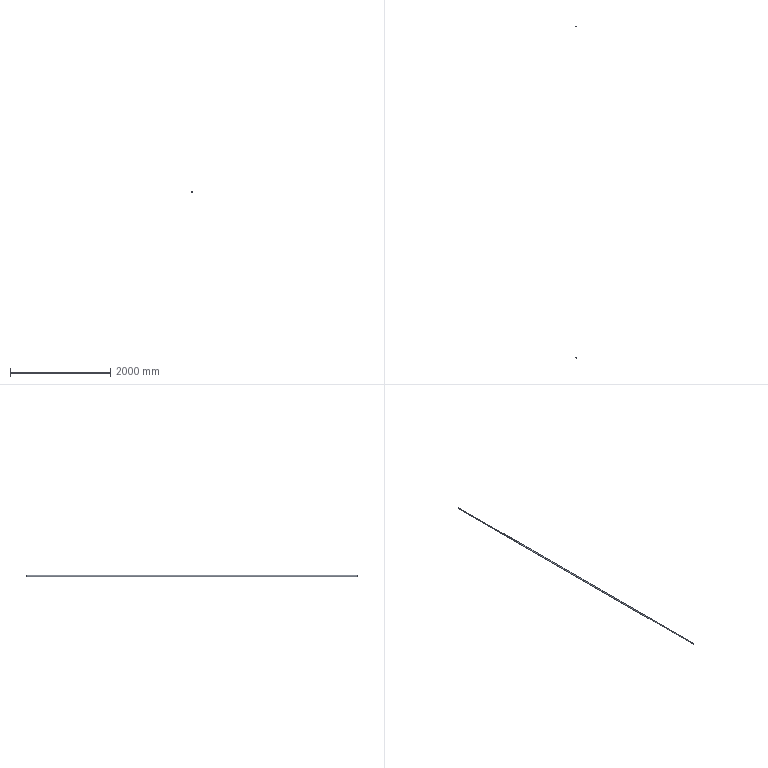Component | NX | 44_7_3 | 1 solid | 4 faces | volume 749835 mm3 | cylinder 2 | plane 2 | commonest cylinder face diameters 20 x1 16 x1